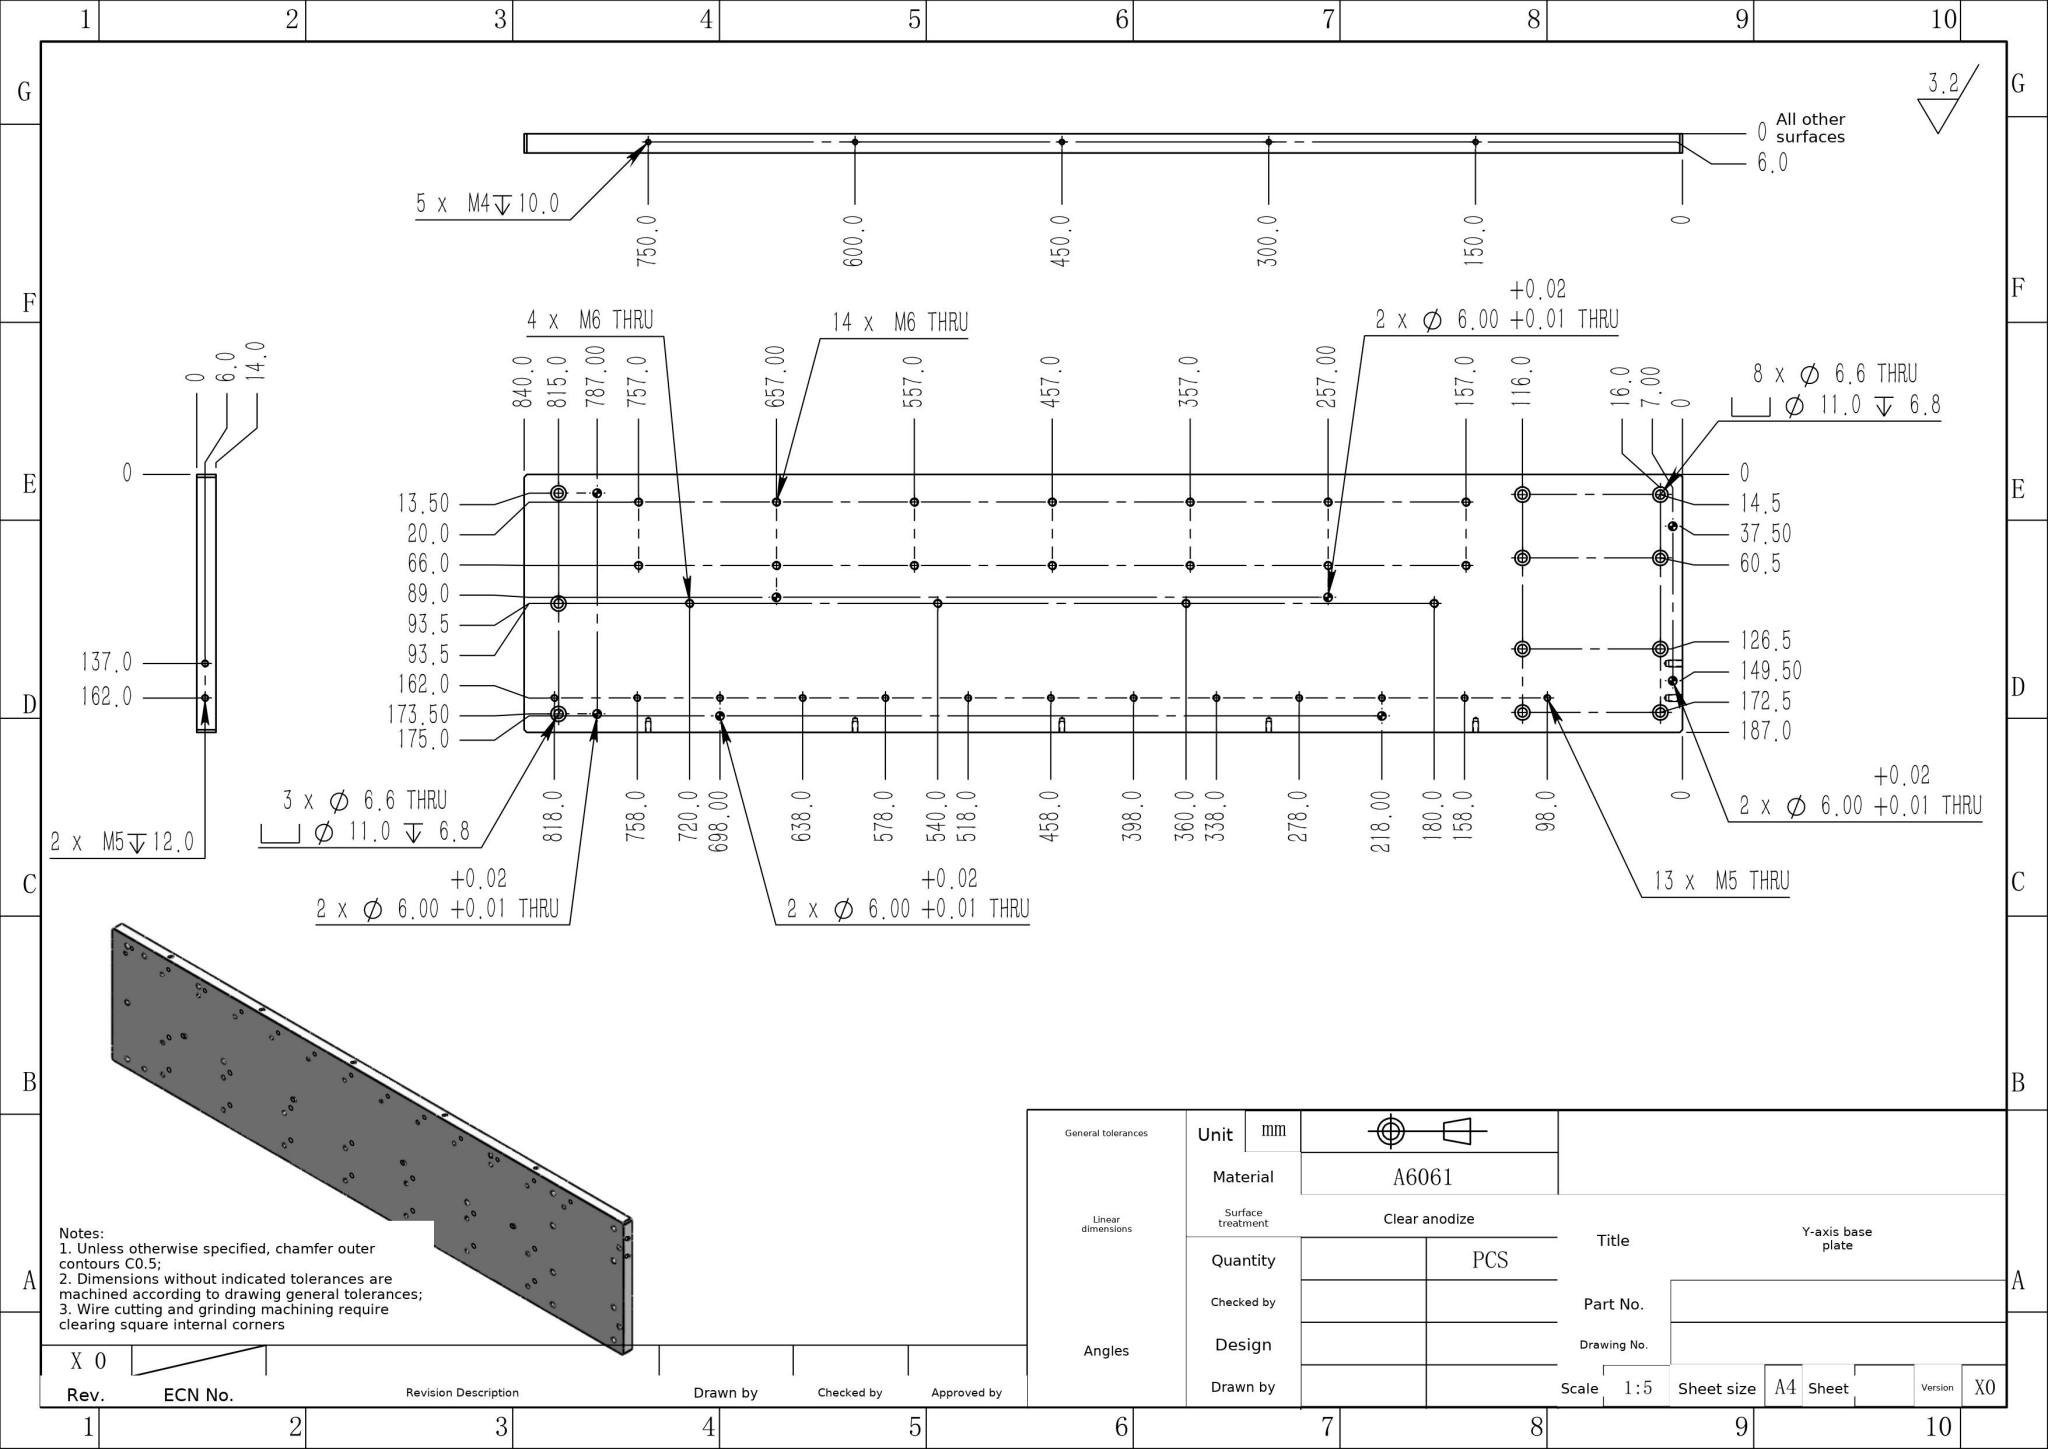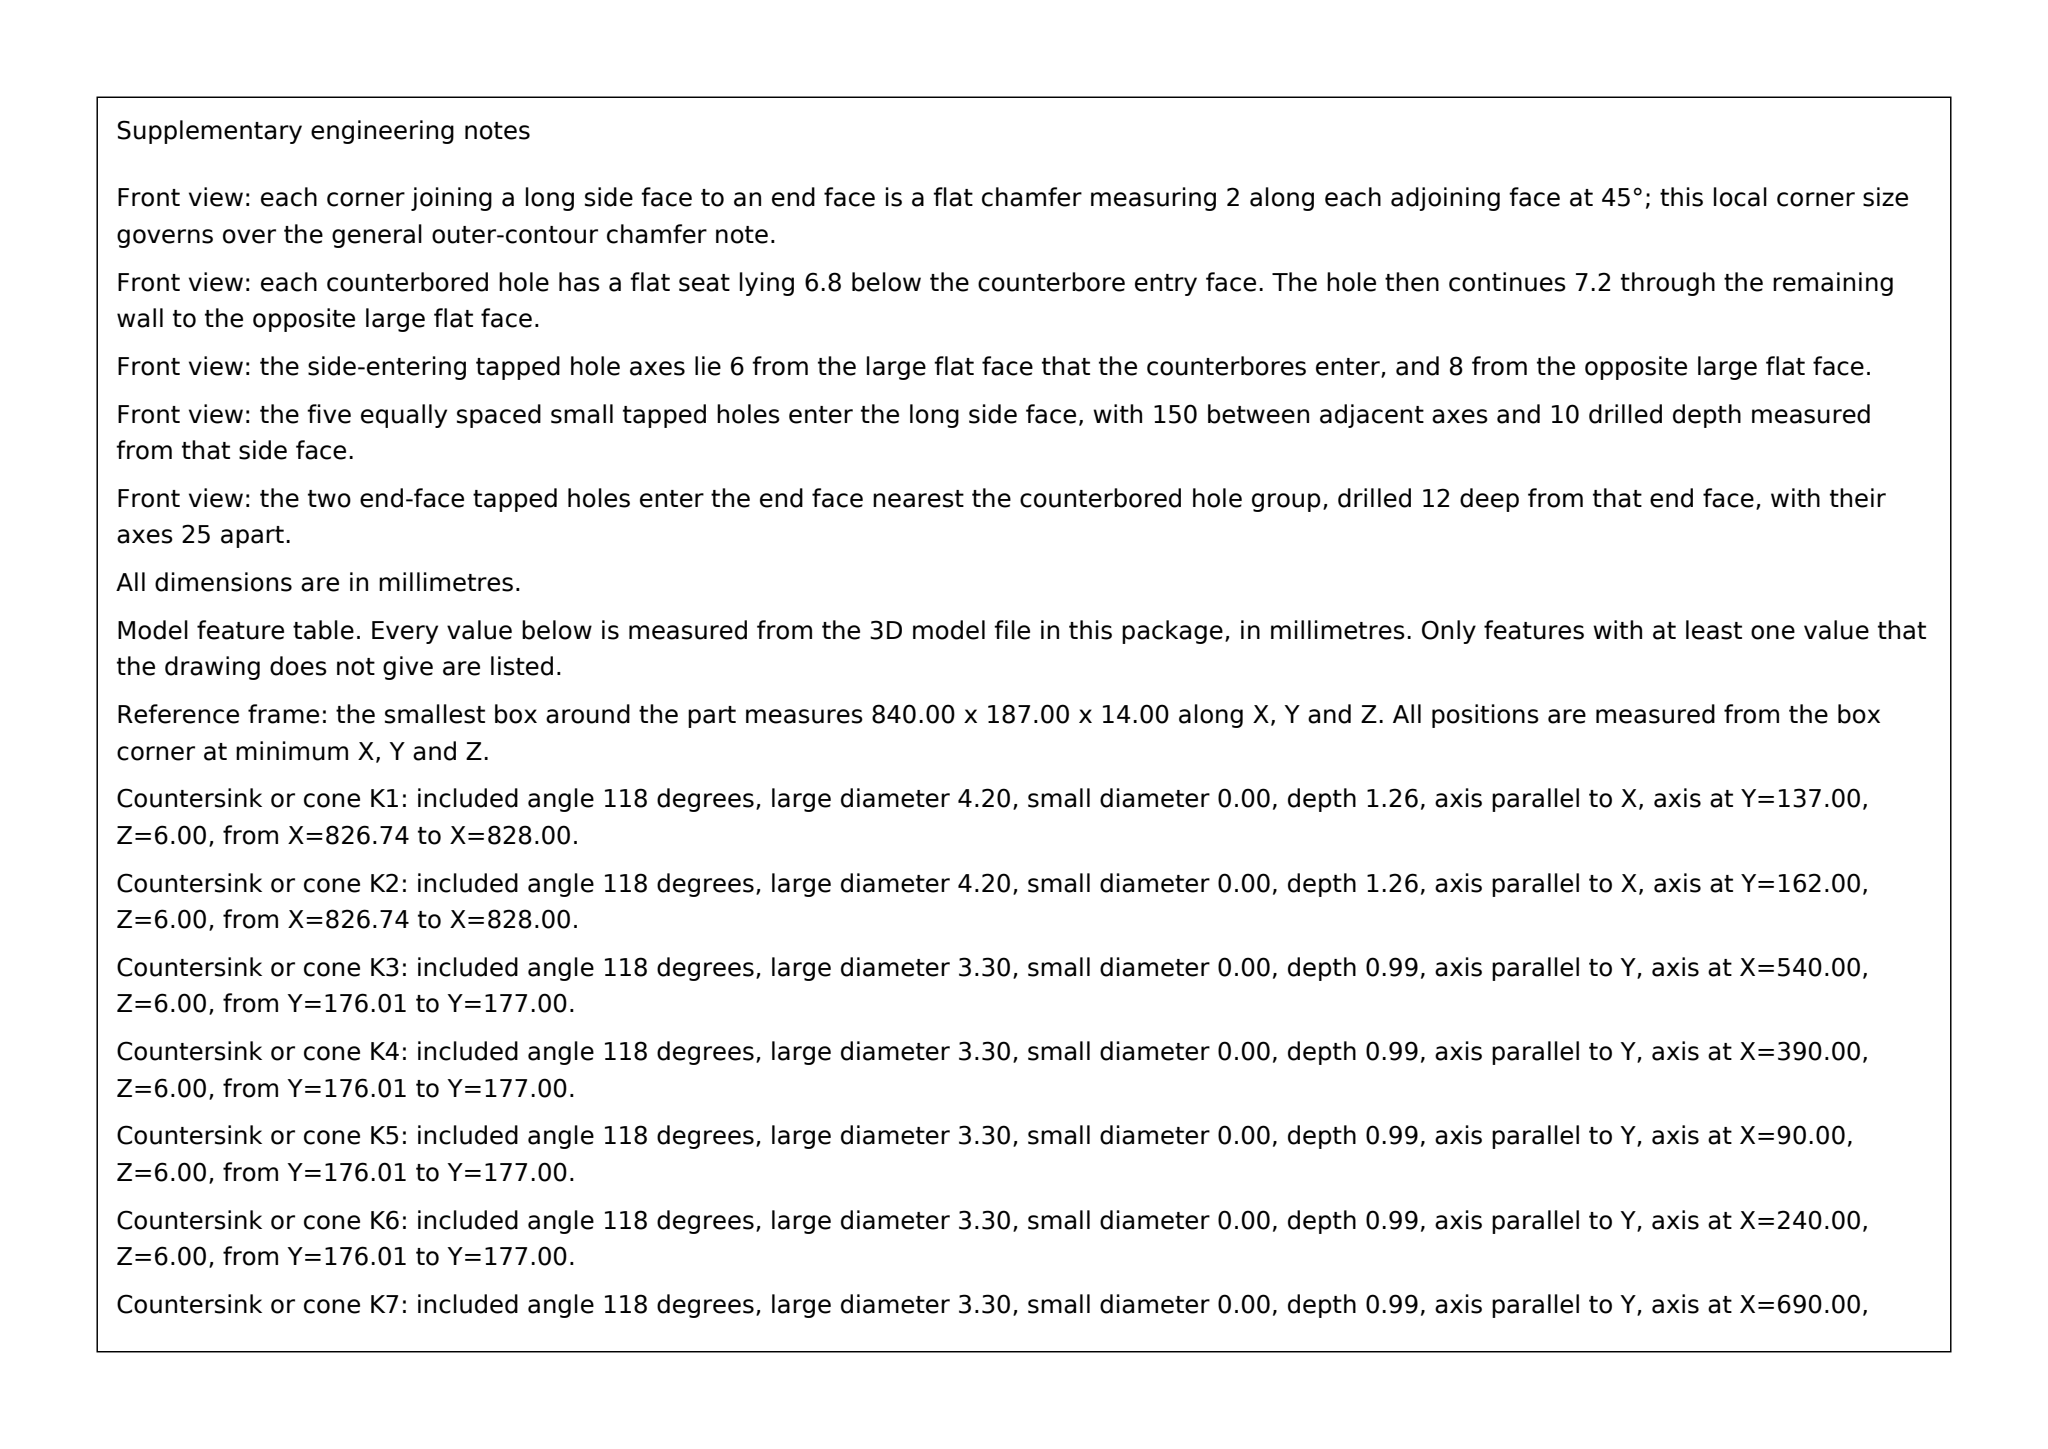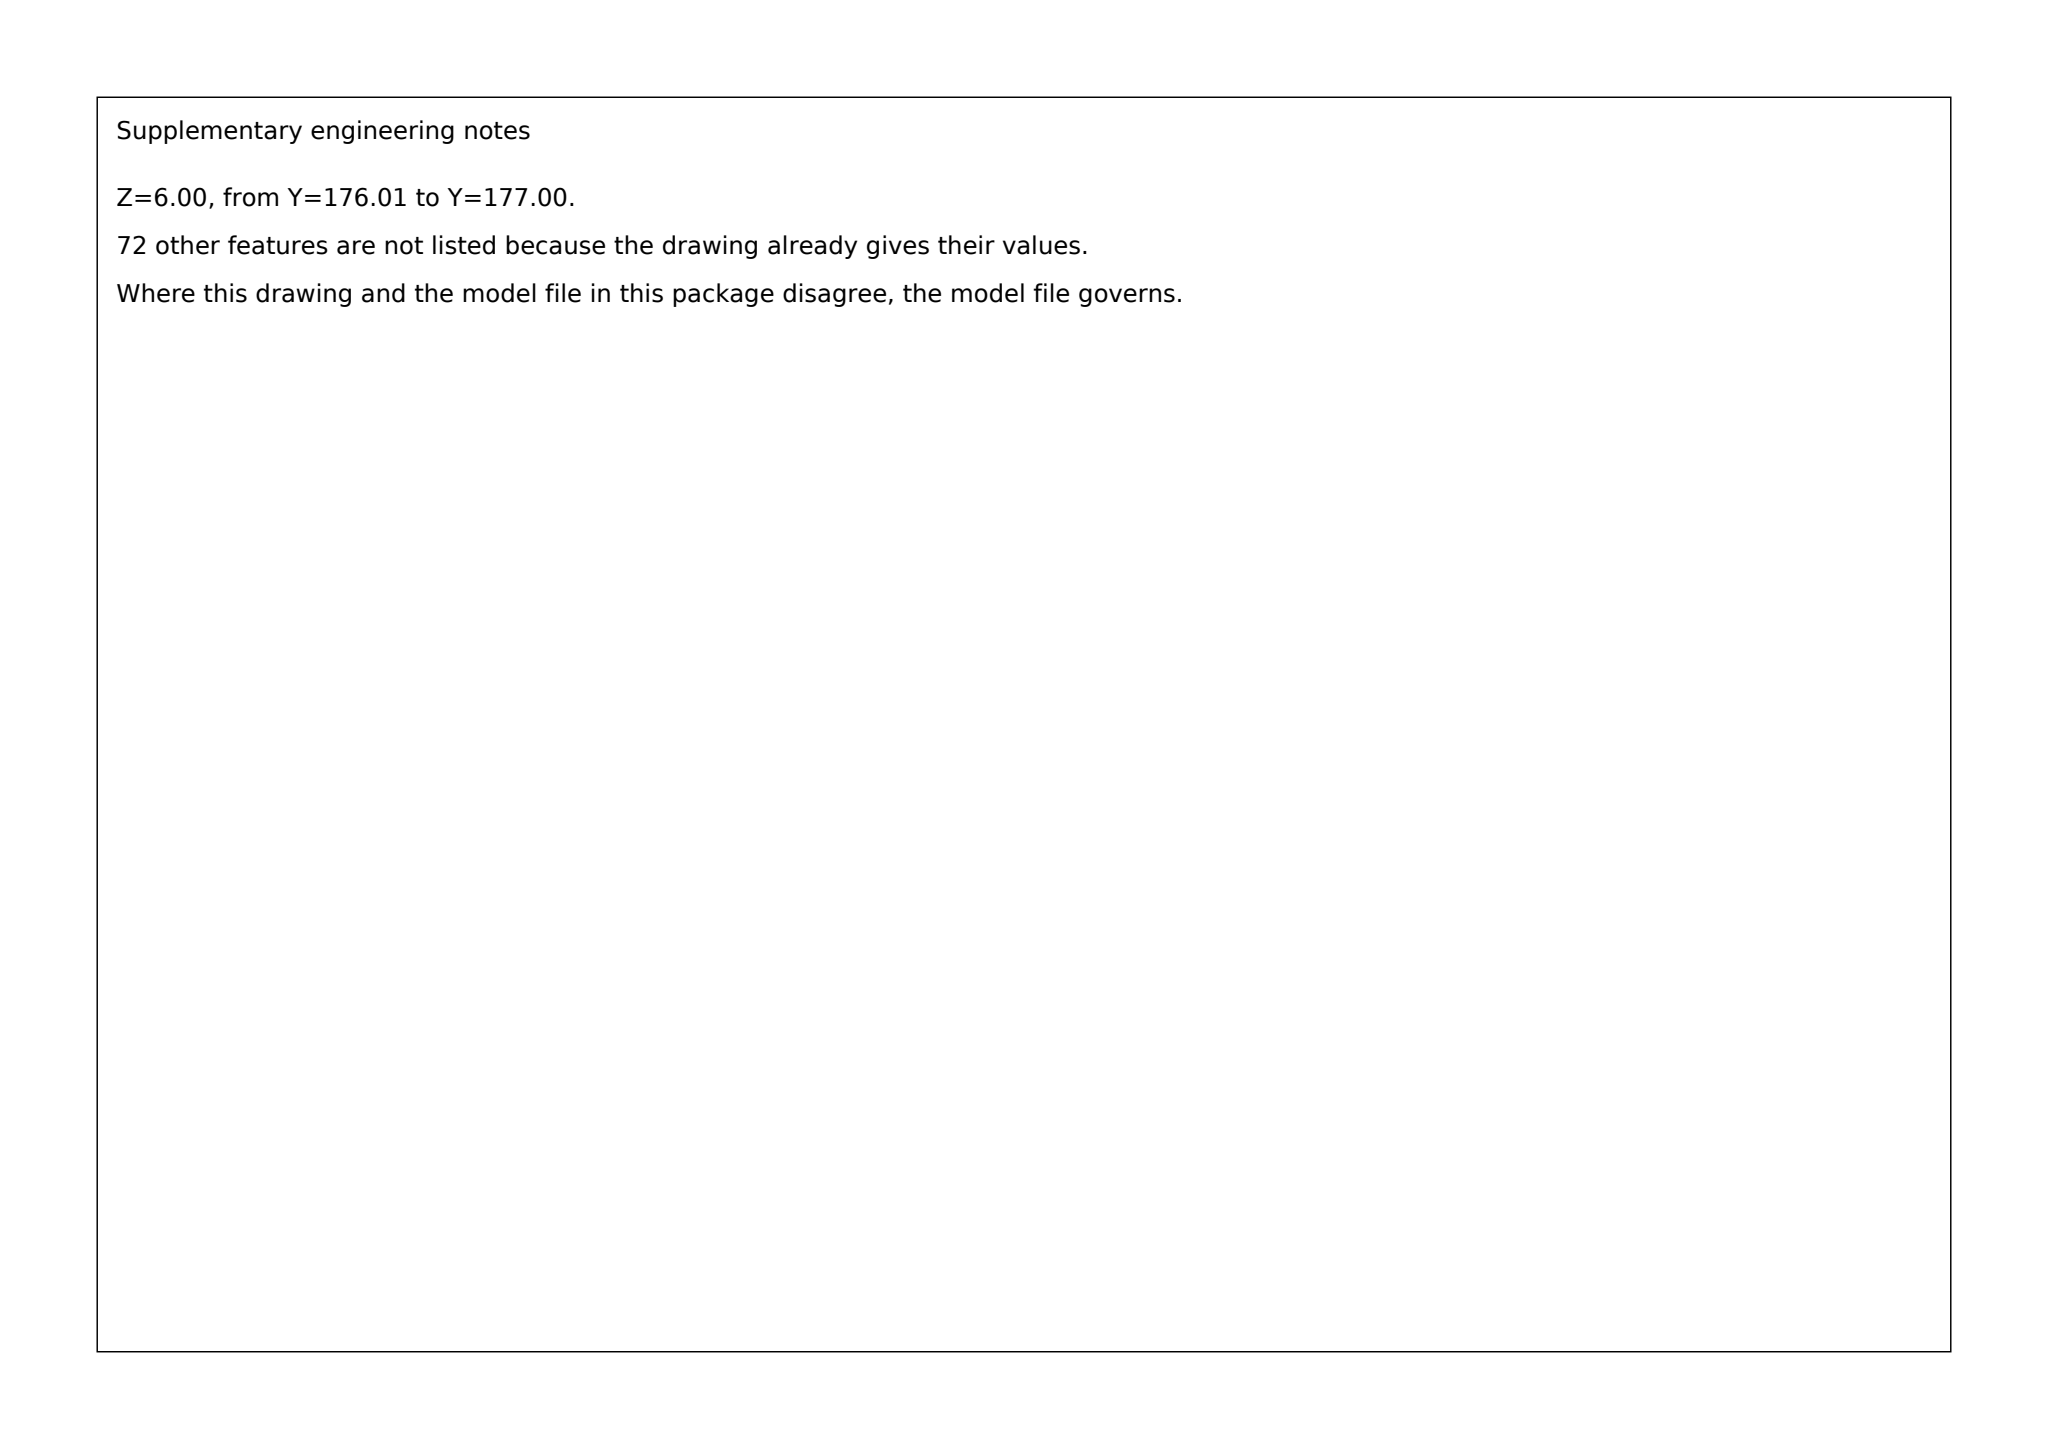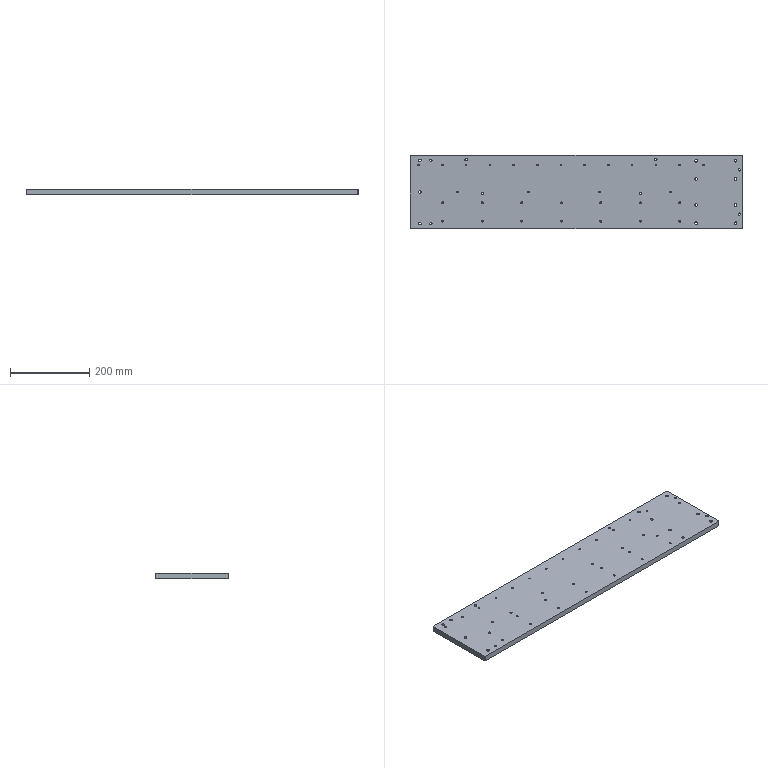Part | SolidWorks | mm | material A6061 | 1 solid | 171 faces | box 840 x 187 x 14 mm | volume 2177768 mm3 | cylinder 136 | plane 21 | cone 14 | commonest cylinder face diameters 5 x36 4.2 x30 11 x22 6.6 x22 6 x16 3.3 x10
build123d program:
from build123d import *

# Parameters (mm, degrees)
SKETCH1_W                                          = 840
SKETCH1_H                                          = 187
BOSS_EXTRUDE1_DEPTH                                = 14
HOLE_SIZE_ACCORDING_TO_TYPE_1_OF_HEXAG_D           = 6.6
HOLE_SIZE_ACCORDING_TO_TYPE_1_OF_HEXAG_CBORE_D     = 11
HOLE_SIZE_ACCORDING_TO_TYPE_1_OF_HEXAG_CBORE_DEPTH = 6.8
SIZE_MM_DOWEL_PIN_HOLE_1_D                         = 6
M6_TAPPED_HOLE1_D                                  = 5
SIZE_MM_DOWEL_PIN_HOLE_3_D                         = 6
M6_TAPPED_HOLE2_D                                  = 5
HOLE_SIZE_ACCORDING_TO_TYPE_2_OF_HEXAG_D           = 6.6
HOLE_SIZE_ACCORDING_TO_TYPE_2_OF_HEXAG_CBORE_D     = 11
HOLE_SIZE_ACCORDING_TO_TYPE_2_OF_HEXAG_CBORE_DEPTH = 6.8
SIZE_MM_DOWEL_PIN_HOLE_2_D                         = 6
M5_TAPPED_HOLE2_D                                  = 4.2
M4_TAPPED_HOLE1_D                                  = 3.3
M4_TAPPED_HOLE1_DEPTH                              = 10
M4_TAPPED_HOLE1_TIP                                = 0.9914
SIZE_MM_DOWEL_PIN_HOLE_4_D                         = 6
M5_TAPPED_HOLE4_D                                  = 4.2
M5_TAPPED_HOLE4_DEPTH                              = 12
M5_TAPPED_HOLE4_TIP                                = 1.262
CHAMFER1_SIZE                                      = 2


with BuildPart() as part:
    # Sketch1 → Boss-Extrude1 (new body)
    with BuildSketch(Plane.XY):
        Rectangle(SKETCH1_W, SKETCH1_H)
    extrude(amount=BOSS_EXTRUDE1_DEPTH)

    # Hole Size _According to_ Type 1 of Hexag (through all)
    with Locations(Plane(origin=(0, 0, 0), x_dir=(-1, 0, 0), z_dir=(0, 0, -1))):
        with Locations((-304, -33), (-304, -79), (-404, -79), (-404, -33), (-404, 33), (-404, 79), (-304, 79), (-304, 33)):
            CounterBoreHole(HOLE_SIZE_ACCORDING_TO_TYPE_1_OF_HEXAG_D / 2, HOLE_SIZE_ACCORDING_TO_TYPE_1_OF_HEXAG_CBORE_D / 2, HOLE_SIZE_ACCORDING_TO_TYPE_1_OF_HEXAG_CBORE_DEPTH)

    # Size mm Dowel Pin Hole 1 (through all)
    with Locations(Plane(origin=(0, 0, 0), x_dir=(-1, 0, 0), z_dir=(0, 0, -1))):
        with Locations((-413, -56), (-413, 56)):
            Hole(SIZE_MM_DOWEL_PIN_HOLE_1_D / 2)

    # M6 Tapped Hole1 (through all)
    with Locations(Plane(origin=(0, 0, 0), x_dir=(-1, 0, 0), z_dir=(0, 0, -1))):
        with Locations((337, -27.5), (337, -73.5), (237, -27.5), (237, -73.5), (137, -27.5), (137, -73.5), (37, -27.5), (37, -73.5), (-63, -27.5), (-63, -73.5), (-163, -27.5), (-163, -73.5), (-263, -27.5), (-263, -73.5)):
            Hole(M6_TAPPED_HOLE1_D / 2)

    # Size mm Dowel Pin Hole 3 (through all)
    with Locations(Plane(origin=(0, 0, 0), x_dir=(-1, 0, 0), z_dir=(0, 0, -1))):
        with Locations((237, -4.5), (-163, -4.5)):
            Hole(SIZE_MM_DOWEL_PIN_HOLE_3_D / 2)

    # M6 Tapped Hole2 (through all)
    with Locations(Plane.XY.offset(14)):
        with Locations((240, 0), (60, 0), (-120, 0), (-300, 0)):
            Hole(M6_TAPPED_HOLE2_D / 2)

    # Hole Size _According to_ Type 2 of Hexag (through all)
    with Locations(Plane(origin=(0, 0, 0), x_dir=(-1, 0, 0), z_dir=(0, 0, -1))):
        with Locations((395, 80), (395, 0), (395, -80)):
            CounterBoreHole(HOLE_SIZE_ACCORDING_TO_TYPE_2_OF_HEXAG_D / 2, HOLE_SIZE_ACCORDING_TO_TYPE_2_OF_HEXAG_CBORE_D / 2, HOLE_SIZE_ACCORDING_TO_TYPE_2_OF_HEXAG_CBORE_DEPTH)

    # Size mm Dowel Pin Hole 2 (through all)
    with Locations(Plane(origin=(0, 0, 0), x_dir=(-1, 0, 0), z_dir=(0, 0, -1))):
        with Locations((367, -80), (367, 80)):
            Hole(SIZE_MM_DOWEL_PIN_HOLE_2_D / 2)

    # M5 Tapped Hole2 (through all)
    with Locations(Plane(origin=(0, 0, 0), x_dir=(-1, 0, 0), z_dir=(0, 0, -1))):
        with Locations((-322, 68.5), (-262, 68.5), (-202, 68.5), (-142, 68.5), (-82, 68.5), (-22, 68.5), (38, 68.5), (98, 68.5), (158, 68.5), (218, 68.5), (278, 68.5), (338, 68.5), (398, 68.5)):
            Hole(M5_TAPPED_HOLE2_D / 2)

    # M4 Tapped Hole1
    with Locations(Plane(origin=(0, 93.5, 0), x_dir=(1, 0, 0), z_dir=(0, 1, 0))):
        with Locations((-330, -6), (-180, -6), (-30, -6), (120, -6), (270, -6)):
            Hole(M4_TAPPED_HOLE1_D / 2, depth=M4_TAPPED_HOLE1_DEPTH)
            with Locations((0, 0, -(M4_TAPPED_HOLE1_DEPTH + M4_TAPPED_HOLE1_TIP / 2))):  # 118° drill point
                Cone(0, M4_TAPPED_HOLE1_D / 2, M4_TAPPED_HOLE1_TIP, mode=Mode.SUBTRACT)

    # Size mm Dowel Pin Hole 4 (through all)
    with Locations(Plane(origin=(0, 0, 0), x_dir=(-1, 0, 0), z_dir=(0, 0, -1))):
        with Locations((278, 81.5), (-202, 81.5)):
            Hole(SIZE_MM_DOWEL_PIN_HOLE_4_D / 2)

    # M5 Tapped Hole4
    with Locations(Plane(origin=(420, 0, 0), x_dir=(0, 0, -1), z_dir=(1, 0, 0))):
        with Locations((-6, 68.5), (-6, 43.5)):
            Hole(M5_TAPPED_HOLE4_D / 2, depth=M5_TAPPED_HOLE4_DEPTH)
            with Locations((0, 0, -(M5_TAPPED_HOLE4_DEPTH + M5_TAPPED_HOLE4_TIP / 2))):  # 118° drill point
                Cone(0, M5_TAPPED_HOLE4_D / 2, M5_TAPPED_HOLE4_TIP, mode=Mode.SUBTRACT)

    # Chamfer1
    chamfer1_edges = [part.edges().sort_by_distance(p)[0] for p in [
        (420, -93.5, 7),
        (-420, -93.5, 7),
        (-420, 93.5, 7),
        (420, 93.5, 7),
    ]]
    chamfer(chamfer1_edges, length=CHAMFER1_SIZE)


solid = part.part